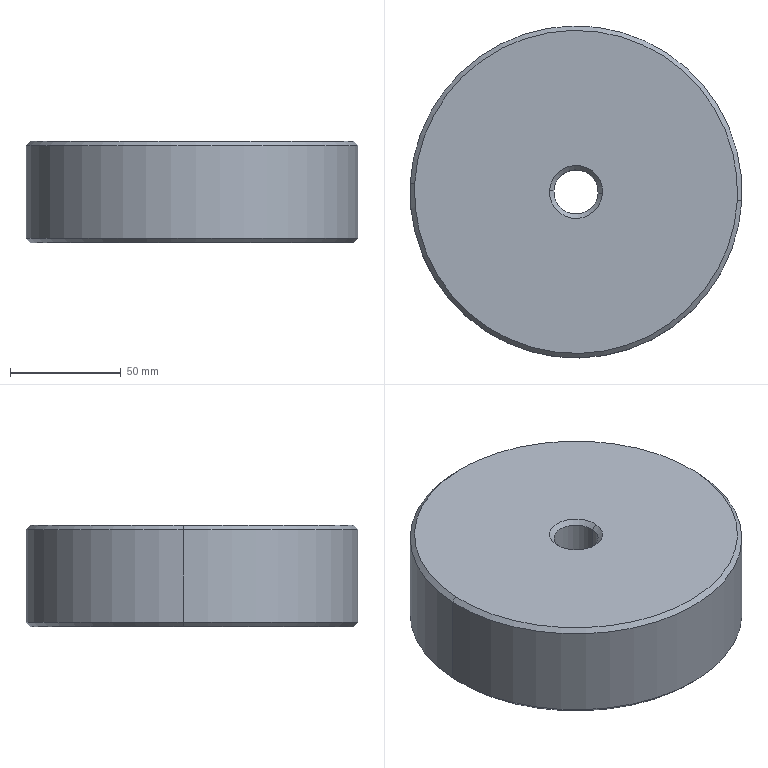Component | SolidWorks | cz-1 | 1 solid | 14 faces | box 150 x 150 x 46 mm | volume 796299 mm3 | cone 8 | cylinder 4 | plane 2 | commonest cylinder face diameters 20 x2 150 x2
build123d program:
from build123d import *

# Parameters (mm, degrees)
SKETCH1_R           = 75
SKETCH1_R_2         = 10
BOSS_EXTRUDE1_DEPTH = 23
CHAMFER1_SIZE       = 2


with BuildPart() as part:
    # Sketch1 → Boss-Extrude1 (new, symmetric)
    with BuildSketch(Plane.XY):
        Circle(SKETCH1_R)
        Circle(SKETCH1_R_2, mode=Mode.SUBTRACT)
    extrude(amount=BOSS_EXTRUDE1_DEPTH, both=True)

    # Chamfer1
    chamfer1_edges = [part.edges().sort_by_distance(p)[0] for p in [
        (-75, 0, -23),
        (-75, 0, 23),
        (-10, 0, -23),
        (-10, 0, 23),
    ]]
    chamfer(chamfer1_edges, length=CHAMFER1_SIZE)


solid = part.part

# Placed as in the assembly
solid = solid.moved(Location((997.956, -215.048, 442), (0, 0, 0)))
STEP:
#1=CARTESIAN_POINT('',(36.42,-8.313,18.307));
#2=VERTEX_POINT('',#1);
#3=CARTESIAN_POINT('',(42.16,-8.62,18.307));
#4=VERTEX_POINT('',#3);
#5=CARTESIAN_POINT('',(39.29,-8.466,18.307));
#6=DIRECTION('',(-0.,-0.,1.));
#7=DIRECTION('',(-0.9986,0.0534,0.));
#8=AXIS2_PLACEMENT_3D('',#5,#6,#7);
#9=CIRCLE('',#8,2.874);
#10=EDGE_CURVE('',#2,#4,#9,.T.);
#11=ORIENTED_EDGE('',*,*,#10,.F.);
#12=CARTESIAN_POINT('',(36.341,-8.309,18.228));
#13=VERTEX_POINT('',#12);
#14=CARTESIAN_POINT('',(36.42,-8.313,18.307));
#15=DIRECTION('',(-0.7061,0.03776,-0.7071));
#16=VECTOR('',#15,39.37);
#17=LINE('',#14,#16);
#18=EDGE_CURVE('',#2,#13,#17,.T.);
#19=ORIENTED_EDGE('',*,*,#18,.T.);
#20=CARTESIAN_POINT('',(42.238,-8.624,18.228));
#21=VERTEX_POINT('',#20);
#22=CARTESIAN_POINT('',(39.29,-8.466,18.228));
#23=DIRECTION('',(0.,0.,-1.));
#24=DIRECTION('',(-0.9986,0.0534,0.));
#25=AXIS2_PLACEMENT_3D('',#22,#23,#24);
#26=CIRCLE('',#25,2.953);
#27=EDGE_CURVE('',#21,#13,#26,.T.);
#28=ORIENTED_EDGE('',*,*,#27,.F.);
#29=CARTESIAN_POINT('',(42.16,-8.62,18.307));
#30=DIRECTION('',(0.7061,-0.03776,-0.7071));
#31=VECTOR('',#30,39.37);
#32=LINE('',#29,#31);
#33=EDGE_CURVE('',#4,#21,#32,.T.);
#34=ORIENTED_EDGE('',*,*,#33,.F.);
#35=EDGE_LOOP('',(#11,#19,#28,#34));
#36=FACE_OUTER_BOUND('',#35,.T.);
#37=CARTESIAN_POINT('',(39.29,-8.466,18.307));
#38=DIRECTION('',(0.,0.,-1.));
#39=DIRECTION('',(0.9986,-0.0534,0.));
#40=AXIS2_PLACEMENT_3D('',#37,#38,#39);
#41=CONICAL_SURFACE('',#40,2.874,0.7854);
#42=ADVANCED_FACE('',(#36),#41,.T.);
#43=CARTESIAN_POINT('',(39.683,-8.487,18.228));
#44=VERTEX_POINT('',#43);
#45=CARTESIAN_POINT('',(38.896,-8.445,18.228));
#46=VERTEX_POINT('',#45);
#47=CARTESIAN_POINT('',(39.29,-8.466,18.228));
#48=DIRECTION('',(-0.,-0.,1.));
#49=DIRECTION('',(-0.9986,0.0534,0.));
#50=AXIS2_PLACEMENT_3D('',#47,#48,#49);
#51=CIRCLE('',#50,0.3937);
#52=EDGE_CURVE('',#44,#46,#51,.T.);
#53=ORIENTED_EDGE('',*,*,#52,.F.);
#54=CARTESIAN_POINT('',(39.761,-8.492,18.307));
#55=VERTEX_POINT('',#54);
#56=CARTESIAN_POINT('',(39.683,-8.487,18.228));
#57=DIRECTION('',(0.7061,-0.03776,0.7071));
#58=VECTOR('',#57,39.37);
#59=LINE('',#56,#58);
#60=EDGE_CURVE('',#44,#55,#59,.T.);
#61=ORIENTED_EDGE('',*,*,#60,.T.);
#62=CARTESIAN_POINT('',(38.818,-8.441,18.307));
#63=VERTEX_POINT('',#62);
#64=CARTESIAN_POINT('',(39.29,-8.466,18.307));
#65=DIRECTION('',(0.,0.,-1.));
#66=DIRECTION('',(-0.9986,0.0534,0.));
#67=AXIS2_PLACEMENT_3D('',#64,#65,#66);
#68=CIRCLE('',#67,0.4724);
#69=EDGE_CURVE('',#63,#55,#68,.T.);
#70=ORIENTED_EDGE('',*,*,#69,.F.);
#71=CARTESIAN_POINT('',(38.896,-8.445,18.228));
#72=DIRECTION('',(-0.7061,0.03776,0.7071));
#73=VECTOR('',#72,39.37);
#74=LINE('',#71,#73);
#75=EDGE_CURVE('',#46,#63,#74,.T.);
#76=ORIENTED_EDGE('',*,*,#75,.F.);
#77=EDGE_LOOP('',(#53,#61,#70,#76));
#78=FACE_OUTER_BOUND('',#77,.T.);
#79=CARTESIAN_POINT('',(39.29,-8.466,18.228));
#80=DIRECTION('',(-0.,-0.,1.));
#81=DIRECTION('',(-0.9986,0.0534,0.));
#82=AXIS2_PLACEMENT_3D('',#79,#80,#81);
#83=CONICAL_SURFACE('',#82,0.3937,0.7854);
#84=ADVANCED_FACE('',(#78),#83,.F.);
#85=CARTESIAN_POINT('',(42.16,-8.62,16.496));
#86=VERTEX_POINT('',#85);
#87=CARTESIAN_POINT('',(36.42,-8.313,16.496));
#88=VERTEX_POINT('',#87);
#89=CARTESIAN_POINT('',(39.29,-8.466,16.496));
#90=DIRECTION('',(0.,0.,-1.));
#91=DIRECTION('',(-0.9986,0.0534,0.));
#92=AXIS2_PLACEMENT_3D('',#89,#90,#91);
#93=CIRCLE('',#92,2.874);
#94=EDGE_CURVE('',#86,#88,#93,.T.);
#95=ORIENTED_EDGE('',*,*,#94,.F.);
#96=CARTESIAN_POINT('',(42.238,-8.624,16.575));
#97=VERTEX_POINT('',#96);
#98=CARTESIAN_POINT('',(42.238,-8.624,16.575));
#99=DIRECTION('',(0.7061,-0.03776,0.7071));
#100=VECTOR('',#99,39.37);
#101=LINE('',#98,#100);
#102=EDGE_CURVE('',#86,#97,#101,.T.);
#103=ORIENTED_EDGE('',*,*,#102,.T.);
#104=CARTESIAN_POINT('',(36.341,-8.309,16.575));
#105=VERTEX_POINT('',#104);
#106=CARTESIAN_POINT('',(39.29,-8.466,16.575));
#107=DIRECTION('',(-0.,-0.,1.));
#108=DIRECTION('',(-0.9986,0.0534,0.));
#109=AXIS2_PLACEMENT_3D('',#106,#107,#108);
#110=CIRCLE('',#109,2.953);
#111=EDGE_CURVE('',#105,#97,#110,.T.);
#112=ORIENTED_EDGE('',*,*,#111,.F.);
#113=CARTESIAN_POINT('',(36.341,-8.309,16.575));
#114=DIRECTION('',(-0.7061,0.03776,0.7071));
#115=VECTOR('',#114,39.37);
#116=LINE('',#113,#115);
#117=EDGE_CURVE('',#88,#105,#116,.T.);
#118=ORIENTED_EDGE('',*,*,#117,.F.);
#119=EDGE_LOOP('',(#95,#103,#112,#118));
#120=FACE_OUTER_BOUND('',#119,.T.);
#121=CARTESIAN_POINT('',(39.29,-8.466,16.575));
#122=DIRECTION('',(-0.,-0.,1.));
#123=DIRECTION('',(-0.9986,0.0534,0.));
#124=AXIS2_PLACEMENT_3D('',#121,#122,#123);
#125=CONICAL_SURFACE('',#124,2.953,0.7854);
#126=ADVANCED_FACE('',(#120),#125,.T.);
#127=CARTESIAN_POINT('',(38.896,-8.445,16.575));
#128=VERTEX_POINT('',#127);
#129=CARTESIAN_POINT('',(39.683,-8.487,16.575));
#130=VERTEX_POINT('',#129);
#131=CARTESIAN_POINT('',(39.29,-8.466,16.575));
#132=DIRECTION('',(0.,0.,-1.));
#133=DIRECTION('',(-0.9986,0.0534,0.));
#134=AXIS2_PLACEMENT_3D('',#131,#132,#133);
#135=CIRCLE('',#134,0.3937);
#136=EDGE_CURVE('',#128,#130,#135,.T.);
#137=ORIENTED_EDGE('',*,*,#136,.F.);
#138=CARTESIAN_POINT('',(38.818,-8.441,16.496));
#139=VERTEX_POINT('',#138);
#140=CARTESIAN_POINT('',(38.818,-8.441,16.496));
#141=DIRECTION('',(-0.7061,0.03776,-0.7071));
#142=VECTOR('',#141,39.37);
#143=LINE('',#140,#142);
#144=EDGE_CURVE('',#128,#139,#143,.T.);
#145=ORIENTED_EDGE('',*,*,#144,.T.);
#146=CARTESIAN_POINT('',(39.761,-8.492,16.496));
#147=VERTEX_POINT('',#146);
#148=CARTESIAN_POINT('',(39.29,-8.466,16.496));
#149=DIRECTION('',(-0.,-0.,1.));
#150=DIRECTION('',(-0.9986,0.0534,0.));
#151=AXIS2_PLACEMENT_3D('',#148,#149,#150);
#152=CIRCLE('',#151,0.4724);
#153=EDGE_CURVE('',#147,#139,#152,.T.);
#154=ORIENTED_EDGE('',*,*,#153,.F.);
#155=CARTESIAN_POINT('',(39.761,-8.492,16.496));
#156=DIRECTION('',(0.7061,-0.03776,-0.7071));
#157=VECTOR('',#156,39.37);
#158=LINE('',#155,#157);
#159=EDGE_CURVE('',#130,#147,#158,.T.);
#160=ORIENTED_EDGE('',*,*,#159,.F.);
#161=EDGE_LOOP('',(#137,#145,#154,#160));
#162=FACE_OUTER_BOUND('',#161,.T.);
#163=CARTESIAN_POINT('',(39.29,-8.466,16.496));
#164=DIRECTION('',(0.,0.,-1.));
#165=DIRECTION('',(0.9986,-0.0534,0.));
#166=AXIS2_PLACEMENT_3D('',#163,#164,#165);
#167=CONICAL_SURFACE('',#166,0.4724,0.7854);
#168=ADVANCED_FACE('',(#162),#167,.F.);
#169=ORIENTED_EDGE('',*,*,#52,.T.);
#170=CARTESIAN_POINT('',(38.896,-8.445,18.307));
#171=DIRECTION('',(0.,0.,-1.));
#172=VECTOR('',#171,39.37);
#173=LINE('',#170,#172);
#174=EDGE_CURVE('',#46,#128,#173,.T.);
#175=ORIENTED_EDGE('',*,*,#174,.T.);
#176=ORIENTED_EDGE('',*,*,#136,.T.);
#177=CARTESIAN_POINT('',(39.683,-8.487,18.307));
#178=DIRECTION('',(0.,0.,-1.));
#179=VECTOR('',#178,39.37);
#180=LINE('',#177,#179);
#181=EDGE_CURVE('',#44,#130,#180,.T.);
#182=ORIENTED_EDGE('',*,*,#181,.F.);
#183=EDGE_LOOP('',(#169,#175,#176,#182));
#184=FACE_OUTER_BOUND('',#183,.T.);
#185=CARTESIAN_POINT('',(39.29,-8.466,18.307));
#186=DIRECTION('',(0.,0.,-1.));
#187=DIRECTION('',(0.9986,-0.0534,0.));
#188=AXIS2_PLACEMENT_3D('',#185,#186,#187);
#189=CYLINDRICAL_SURFACE('',#188,0.3937);
#190=ADVANCED_FACE('',(#184),#189,.F.);
#191=ORIENTED_EDGE('',*,*,#27,.T.);
#192=CARTESIAN_POINT('',(36.341,-8.309,18.307));
#193=DIRECTION('',(0.,0.,-1.));
#194=VECTOR('',#193,39.37);
#195=LINE('',#192,#194);
#196=EDGE_CURVE('',#13,#105,#195,.T.);
#197=ORIENTED_EDGE('',*,*,#196,.T.);
#198=ORIENTED_EDGE('',*,*,#111,.T.);
#199=CARTESIAN_POINT('',(42.238,-8.624,18.307));
#200=DIRECTION('',(0.,0.,-1.));
#201=VECTOR('',#200,39.37);
#202=LINE('',#199,#201);
#203=EDGE_CURVE('',#21,#97,#202,.T.);
#204=ORIENTED_EDGE('',*,*,#203,.F.);
#205=EDGE_LOOP('',(#191,#197,#198,#204));
#206=FACE_OUTER_BOUND('',#205,.T.);
#207=CARTESIAN_POINT('',(39.29,-8.466,18.307));
#208=DIRECTION('',(0.,0.,-1.));
#209=DIRECTION('',(0.9986,-0.0534,0.));
#210=AXIS2_PLACEMENT_3D('',#207,#208,#209);
#211=CYLINDRICAL_SURFACE('',#210,2.953);
#212=ADVANCED_FACE('',(#206),#211,.T.);
#213=ORIENTED_EDGE('',*,*,#69,.T.);
#214=CARTESIAN_POINT('',(39.29,-8.466,18.307));
#215=DIRECTION('',(0.,0.,-1.));
#216=DIRECTION('',(-0.9986,0.0534,0.));
#217=AXIS2_PLACEMENT_3D('',#214,#215,#216);
#218=CIRCLE('',#217,0.4724);
#219=EDGE_CURVE('',#55,#63,#218,.T.);
#220=ORIENTED_EDGE('',*,*,#219,.T.);
#221=EDGE_LOOP('',(#213,#220));
#222=FACE_BOUND('',#221,.T.);
#223=CARTESIAN_POINT('',(39.29,-8.466,18.307));
#224=DIRECTION('',(-0.,-0.,1.));
#225=DIRECTION('',(-0.9986,0.0534,0.));
#226=AXIS2_PLACEMENT_3D('',#223,#224,#225);
#227=CIRCLE('',#226,2.874);
#228=EDGE_CURVE('',#4,#2,#227,.T.);
#229=ORIENTED_EDGE('',*,*,#228,.T.);
#230=ORIENTED_EDGE('',*,*,#10,.T.);
#231=EDGE_LOOP('',(#229,#230));
#232=FACE_OUTER_BOUND('',#231,.T.);
#233=CARTESIAN_POINT('',(39.29,-8.466,18.307));
#234=DIRECTION('',(-0.,-0.,1.));
#235=DIRECTION('',(-0.9986,0.0534,-0.));
#236=AXIS2_PLACEMENT_3D('',#233,#234,#235);
#237=PLANE('',#236);
#238=ADVANCED_FACE('',(#222,#232),#237,.T.);
#239=ORIENTED_EDGE('',*,*,#153,.T.);
#240=CARTESIAN_POINT('',(39.29,-8.466,16.496));
#241=DIRECTION('',(-0.,-0.,1.));
#242=DIRECTION('',(-0.9986,0.0534,0.));
#243=AXIS2_PLACEMENT_3D('',#240,#241,#242);
#244=CIRCLE('',#243,0.4724);
#245=EDGE_CURVE('',#139,#147,#244,.T.);
#246=ORIENTED_EDGE('',*,*,#245,.T.);
#247=EDGE_LOOP('',(#239,#246));
#248=FACE_BOUND('',#247,.T.);
#249=CARTESIAN_POINT('',(39.29,-8.466,16.496));
#250=DIRECTION('',(0.,0.,-1.));
#251=DIRECTION('',(-0.9986,0.0534,0.));
#252=AXIS2_PLACEMENT_3D('',#249,#250,#251);
#253=CIRCLE('',#252,2.874);
#254=EDGE_CURVE('',#88,#86,#253,.T.);
#255=ORIENTED_EDGE('',*,*,#254,.T.);
#256=ORIENTED_EDGE('',*,*,#94,.T.);
#257=EDGE_LOOP('',(#255,#256));
#258=FACE_OUTER_BOUND('',#257,.T.);
#259=CARTESIAN_POINT('',(39.29,-8.466,16.496));
#260=DIRECTION('',(-0.,-0.,1.));
#261=DIRECTION('',(-0.9986,0.0534,-0.));
#262=AXIS2_PLACEMENT_3D('',#259,#260,#261);
#263=PLANE('',#262);
#264=ADVANCED_FACE('',(#248,#258),#263,.F.);
#265=ORIENTED_EDGE('',*,*,#196,.F.);
#266=CARTESIAN_POINT('',(39.29,-8.466,18.228));
#267=DIRECTION('',(0.,0.,-1.));
#268=DIRECTION('',(-0.9986,0.0534,0.));
#269=AXIS2_PLACEMENT_3D('',#266,#267,#268);
#270=CIRCLE('',#269,2.953);
#271=EDGE_CURVE('',#13,#21,#270,.T.);
#272=ORIENTED_EDGE('',*,*,#271,.T.);
#273=ORIENTED_EDGE('',*,*,#203,.T.);
#274=CARTESIAN_POINT('',(39.29,-8.466,16.575));
#275=DIRECTION('',(-0.,-0.,1.));
#276=DIRECTION('',(-0.9986,0.0534,0.));
#277=AXIS2_PLACEMENT_3D('',#274,#275,#276);
#278=CIRCLE('',#277,2.953);
#279=EDGE_CURVE('',#97,#105,#278,.T.);
#280=ORIENTED_EDGE('',*,*,#279,.T.);
#281=EDGE_LOOP('',(#265,#272,#273,#280));
#282=FACE_OUTER_BOUND('',#281,.T.);
#283=CARTESIAN_POINT('',(39.29,-8.466,18.307));
#284=DIRECTION('',(0.,0.,-1.));
#285=DIRECTION('',(0.9986,-0.0534,0.));
#286=AXIS2_PLACEMENT_3D('',#283,#284,#285);
#287=CYLINDRICAL_SURFACE('',#286,2.953);
#288=ADVANCED_FACE('',(#282),#287,.T.);
#289=ORIENTED_EDGE('',*,*,#174,.F.);
#290=CARTESIAN_POINT('',(39.29,-8.466,18.228));
#291=DIRECTION('',(-0.,-0.,1.));
#292=DIRECTION('',(-0.9986,0.0534,0.));
#293=AXIS2_PLACEMENT_3D('',#290,#291,#292);
#294=CIRCLE('',#293,0.3937);
#295=EDGE_CURVE('',#46,#44,#294,.T.);
#296=ORIENTED_EDGE('',*,*,#295,.T.);
#297=ORIENTED_EDGE('',*,*,#181,.T.);
#298=CARTESIAN_POINT('',(39.29,-8.466,16.575));
#299=DIRECTION('',(0.,0.,-1.));
#300=DIRECTION('',(-0.9986,0.0534,0.));
#301=AXIS2_PLACEMENT_3D('',#298,#299,#300);
#302=CIRCLE('',#301,0.3937);
#303=EDGE_CURVE('',#130,#128,#302,.T.);
#304=ORIENTED_EDGE('',*,*,#303,.T.);
#305=EDGE_LOOP('',(#289,#296,#297,#304));
#306=FACE_OUTER_BOUND('',#305,.T.);
#307=CARTESIAN_POINT('',(39.29,-8.466,18.307));
#308=DIRECTION('',(0.,0.,-1.));
#309=DIRECTION('',(0.9986,-0.0534,0.));
#310=AXIS2_PLACEMENT_3D('',#307,#308,#309);
#311=CYLINDRICAL_SURFACE('',#310,0.3937);
#312=ADVANCED_FACE('',(#306),#311,.F.);
#313=ORIENTED_EDGE('',*,*,#144,.F.);
#314=ORIENTED_EDGE('',*,*,#303,.F.);
#315=ORIENTED_EDGE('',*,*,#159,.T.);
#316=ORIENTED_EDGE('',*,*,#245,.F.);
#317=EDGE_LOOP('',(#313,#314,#315,#316));
#318=FACE_OUTER_BOUND('',#317,.T.);
#319=CARTESIAN_POINT('',(39.29,-8.466,16.496));
#320=DIRECTION('',(0.,0.,-1.));
#321=DIRECTION('',(0.9986,-0.0534,0.));
#322=AXIS2_PLACEMENT_3D('',#319,#320,#321);
#323=CONICAL_SURFACE('',#322,0.4724,0.7854);
#324=ADVANCED_FACE('',(#318),#323,.F.);
#325=ORIENTED_EDGE('',*,*,#102,.F.);
#326=ORIENTED_EDGE('',*,*,#254,.F.);
#327=ORIENTED_EDGE('',*,*,#117,.T.);
#328=ORIENTED_EDGE('',*,*,#279,.F.);
#329=EDGE_LOOP('',(#325,#326,#327,#328));
#330=FACE_OUTER_BOUND('',#329,.T.);
#331=CARTESIAN_POINT('',(39.29,-8.466,16.575));
#332=DIRECTION('',(-0.,-0.,1.));
#333=DIRECTION('',(-0.9986,0.0534,0.));
#334=AXIS2_PLACEMENT_3D('',#331,#332,#333);
#335=CONICAL_SURFACE('',#334,2.953,0.7854);
#336=ADVANCED_FACE('',(#330),#335,.T.);
#337=ORIENTED_EDGE('',*,*,#60,.F.);
#338=ORIENTED_EDGE('',*,*,#295,.F.);
#339=ORIENTED_EDGE('',*,*,#75,.T.);
#340=ORIENTED_EDGE('',*,*,#219,.F.);
#341=EDGE_LOOP('',(#337,#338,#339,#340));
#342=FACE_OUTER_BOUND('',#341,.T.);
#343=CARTESIAN_POINT('',(39.29,-8.466,18.228));
#344=DIRECTION('',(-0.,-0.,1.));
#345=DIRECTION('',(-0.9986,0.0534,0.));
#346=AXIS2_PLACEMENT_3D('',#343,#344,#345);
#347=CONICAL_SURFACE('',#346,0.3937,0.7854);
#348=ADVANCED_FACE('',(#342),#347,.F.);
#349=ORIENTED_EDGE('',*,*,#18,.F.);
#350=ORIENTED_EDGE('',*,*,#228,.F.);
#351=ORIENTED_EDGE('',*,*,#33,.T.);
#352=ORIENTED_EDGE('',*,*,#271,.F.);
#353=EDGE_LOOP('',(#349,#350,#351,#352));
#354=FACE_OUTER_BOUND('',#353,.T.);
#355=CARTESIAN_POINT('',(39.29,-8.466,18.307));
#356=DIRECTION('',(0.,0.,-1.));
#357=DIRECTION('',(0.9986,-0.0534,0.));
#358=AXIS2_PLACEMENT_3D('',#355,#356,#357);
#359=CONICAL_SURFACE('',#358,2.874,0.7854);
#360=ADVANCED_FACE('',(#354),#359,.T.);
#361=CLOSED_SHELL('',(#42,#84,#126,#168,#190,#212,#238,#264,#288,#312,#324,#336,#348,#360));
#362=MANIFOLD_SOLID_BREP('',#361);
#363=CARTESIAN_POINT('',(0.,0.,0.));
#364=DIRECTION('',(0.,0.,1.));
#365=DIRECTION('',(1.,0.,0.));
#366=AXIS2_PLACEMENT_3D('',#363,#364,#365);
#367=(LENGTH_UNIT()NAMED_UNIT(*)SI_UNIT($,.METRE.));
#368=LENGTH_MEASURE_WITH_UNIT(LENGTH_MEASURE(0.0254),#367);
#369=DIMENSIONAL_EXPONENTS(1.,0.,0.,0.,0.,0.,0.);
#370=(CONVERSION_BASED_UNIT('',#368)LENGTH_UNIT()NAMED_UNIT(#369));
#371=UNCERTAINTY_MEASURE_WITH_UNIT(LENGTH_MEASURE(0.00001),#370,'','');
#372=(NAMED_UNIT(*)PLANE_ANGLE_UNIT()SI_UNIT($,.RADIAN.));
#373=(NAMED_UNIT(*)SI_UNIT($,.STERADIAN.)SOLID_ANGLE_UNIT());
#374=(GEOMETRIC_REPRESENTATION_CONTEXT(3)GLOBAL_UNCERTAINTY_ASSIGNED_CONTEXT((#371))GLOBAL_UNIT_ASSIGNED_CONTEXT((#370,#372,#373))REPRESENTATION_CONTEXT('',''));
#375=ADVANCED_BREP_SHAPE_REPRESENTATION('',(#362,#366),#374);
#376=COLOUR_RGB('',0.7922,0.8196,0.9333);
#377=FILL_AREA_STYLE_COLOUR('',#376);
#378=FILL_AREA_STYLE('',(#377));
#379=SURFACE_STYLE_FILL_AREA(#378);
#380=SURFACE_SIDE_STYLE('',(#379));
#381=SURFACE_STYLE_USAGE(.BOTH.,#380);
#382=PRESENTATION_STYLE_ASSIGNMENT((#381));
#383=STYLED_ITEM('',(#382),#362);
#384=PRESENTATION_LAYER_ASSIGNMENT('','',(#383));
#385=(LENGTH_UNIT()NAMED_UNIT(*)SI_UNIT($,.METRE.));
#386=LENGTH_MEASURE_WITH_UNIT(LENGTH_MEASURE(0.0254),#385);
#387=DIMENSIONAL_EXPONENTS(1.,0.,0.,0.,0.,0.,0.);
#388=(CONVERSION_BASED_UNIT('',#386)LENGTH_UNIT()NAMED_UNIT(#387));
#389=UNCERTAINTY_MEASURE_WITH_UNIT(LENGTH_MEASURE(0.00001),#388,'','');
#390=(NAMED_UNIT(*)PLANE_ANGLE_UNIT()SI_UNIT($,.RADIAN.));
#391=(NAMED_UNIT(*)SI_UNIT($,.STERADIAN.)SOLID_ANGLE_UNIT());
#392=(GEOMETRIC_REPRESENTATION_CONTEXT(3)GLOBAL_UNCERTAINTY_ASSIGNED_CONTEXT((#389))GLOBAL_UNIT_ASSIGNED_CONTEXT((#388,#390,#391))REPRESENTATION_CONTEXT('',''));
#393=MECHANICAL_DESIGN_GEOMETRIC_PRESENTATION_REPRESENTATION('',(#383),#392);